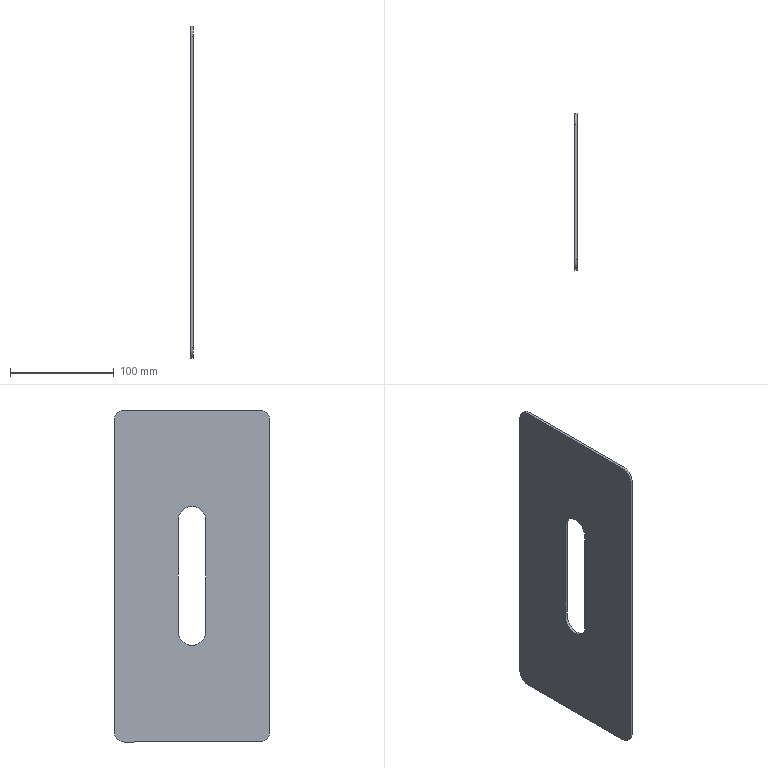Component | SolidWorks | 12ATransverseStraighteningSeatBaffle-1 | 1 solid | 15 faces | box 2.5 x 150.5 x 320.5 mm | volume 111720 mm3 | plane 8 | cylinder 7 | commonest cylinder face diameters 20 x4 27 x3 | material Q235
build123d program:
from build123d import *

# Parameters (mm, degrees)
BOSS_EXTRUDE1_DEPTH = 2.5


with BuildPart() as part:
    # Sketch1 → Boss-Extrude1 (new body)
    with BuildSketch(Plane.XY):
        with BuildLine():
            Line((-150.25, 75.25), (150.25, 75.25))
            ThreePointArc((150.25, 75.25), (157.321, 72.321), (160.25, 65.25))
            Line((160.25, 65.25), (160.25, -65.25))
            ThreePointArc((160.25, -65.25), (157.321, -72.321), (150.25, -75.25))
            Line((150.25, -75.25), (-150.25, -75.25))
            ThreePointArc((-150.25, -75.25), (-157.321, -72.321), (-160.25, -65.25))
            Line((-160.25, -65.25), (-160.25, 65.25))
            ThreePointArc((-160.25, 65.25), (-157.321, 72.321), (-150.25, 75.25))
        make_face()
        with BuildLine():
            Line((-53.5, 13.5), (53.5, 13.5))
            ThreePointArc((53.5, 13.5), (67, 0), (53.5, -13.5))
            Line((53.5, -13.5), (-53.5, -13.5))
            ThreePointArc((-53.5, -13.5), (-67, 0), (-53.5, 13.5))
        make_face(mode=Mode.SUBTRACT)
    extrude(amount=BOSS_EXTRUDE1_DEPTH)


solid = part.part

# Placed as in the assembly
solid = solid.moved(Location((-114.383, 6.96, 31), (0, 90, 0)))
STEP:
#1=COLOUR_RGB('',0.7922,0.8196,0.9333);
#2=FILL_AREA_STYLE_COLOUR('',#1);
#3=FILL_AREA_STYLE('',(#2));
#4=SURFACE_STYLE_FILL_AREA(#3);
#5=SURFACE_SIDE_STYLE('',(#4));
#6=SURFACE_STYLE_USAGE(.BOTH.,#5);
#7=PRESENTATION_STYLE_ASSIGNMENT((#6));
#8=CARTESIAN_POINT('',(-4.405,0.8055,3.327));
#9=VERTEX_POINT('',#8);
#10=CARTESIAN_POINT('',(-4.405,0.274,3.858));
#11=VERTEX_POINT('',#10);
#12=CARTESIAN_POINT('',(-4.405,0.274,3.327));
#13=DIRECTION('',(1.,0.,0.));
#14=DIRECTION('',(0.,-0.,-1.));
#15=AXIS2_PLACEMENT_3D('',#12,#13,#14);
#16=CIRCLE('',#15,0.5315);
#17=EDGE_CURVE('',#9,#11,#16,.T.);
#18=ORIENTED_EDGE('',*,*,#17,.T.);
#19=CARTESIAN_POINT('',(-4.503,0.274,3.858));
#20=VERTEX_POINT('',#19);
#21=CARTESIAN_POINT('',(-4.405,0.274,3.858));
#22=DIRECTION('',(-1.,-0.,0.));
#23=VECTOR('',#22,39.37);
#24=LINE('',#21,#23);
#25=EDGE_CURVE('',#11,#20,#24,.T.);
#26=ORIENTED_EDGE('',*,*,#25,.T.);
#27=CARTESIAN_POINT('',(-4.503,0.8055,3.327));
#28=VERTEX_POINT('',#27);
#29=CARTESIAN_POINT('',(-4.503,0.274,3.327));
#30=DIRECTION('',(1.,0.,0.));
#31=DIRECTION('',(0.,-0.,-1.));
#32=AXIS2_PLACEMENT_3D('',#29,#30,#31);
#33=CIRCLE('',#32,0.5315);
#34=EDGE_CURVE('',#28,#20,#33,.T.);
#35=ORIENTED_EDGE('',*,*,#34,.F.);
#36=CARTESIAN_POINT('',(-4.405,0.8055,3.327));
#37=DIRECTION('',(-1.,-0.,0.));
#38=VECTOR('',#37,39.37);
#39=LINE('',#36,#38);
#40=EDGE_CURVE('',#9,#28,#39,.T.);
#41=ORIENTED_EDGE('',*,*,#40,.F.);
#42=EDGE_LOOP('',(#18,#26,#35,#41));
#43=FACE_OUTER_BOUND('',#42,.T.);
#44=CARTESIAN_POINT('',(-4.405,0.274,3.327));
#45=DIRECTION('',(-1.,-0.,0.));
#46=DIRECTION('',(0.,0.,1.));
#47=AXIS2_PLACEMENT_3D('',#44,#45,#46);
#48=CYLINDRICAL_SURFACE('',#47,0.5315);
#49=ADVANCED_FACE('',(#43),#48,.F.);
#50=CARTESIAN_POINT('',(-4.405,2.843,-5.089));
#51=VERTEX_POINT('',#50);
#52=CARTESIAN_POINT('',(-4.405,3.237,-4.695));
#53=VERTEX_POINT('',#52);
#54=CARTESIAN_POINT('',(-4.405,2.843,-4.695));
#55=DIRECTION('',(1.,0.,0.));
#56=DIRECTION('',(0.,0.,1.));
#57=AXIS2_PLACEMENT_3D('',#54,#55,#56);
#58=CIRCLE('',#57,0.3937);
#59=EDGE_CURVE('',#51,#53,#58,.T.);
#60=ORIENTED_EDGE('',*,*,#59,.T.);
#61=CARTESIAN_POINT('',(-4.405,3.237,7.136));
#62=VERTEX_POINT('',#61);
#63=CARTESIAN_POINT('',(-4.405,3.237,7.136));
#64=DIRECTION('',(-0.,0.,1.));
#65=VECTOR('',#64,39.37);
#66=LINE('',#63,#65);
#67=EDGE_CURVE('',#53,#62,#66,.T.);
#68=ORIENTED_EDGE('',*,*,#67,.T.);
#69=CARTESIAN_POINT('',(-4.405,2.843,7.53));
#70=VERTEX_POINT('',#69);
#71=CARTESIAN_POINT('',(-4.405,2.843,7.136));
#72=DIRECTION('',(1.,0.,0.));
#73=DIRECTION('',(0.,-0.,-1.));
#74=AXIS2_PLACEMENT_3D('',#71,#72,#73);
#75=CIRCLE('',#74,0.3937);
#76=EDGE_CURVE('',#62,#70,#75,.T.);
#77=ORIENTED_EDGE('',*,*,#76,.T.);
#78=CARTESIAN_POINT('',(-4.405,-2.295,7.53));
#79=VERTEX_POINT('',#78);
#80=CARTESIAN_POINT('',(-4.405,2.843,7.53));
#81=DIRECTION('',(0.,-1.,0.));
#82=VECTOR('',#81,39.37);
#83=LINE('',#80,#82);
#84=EDGE_CURVE('',#70,#79,#83,.T.);
#85=ORIENTED_EDGE('',*,*,#84,.T.);
#86=CARTESIAN_POINT('',(-4.405,-2.689,7.136));
#87=VERTEX_POINT('',#86);
#88=CARTESIAN_POINT('',(-4.405,-2.295,7.136));
#89=DIRECTION('',(1.,0.,0.));
#90=DIRECTION('',(0.,-0.,-1.));
#91=AXIS2_PLACEMENT_3D('',#88,#89,#90);
#92=CIRCLE('',#91,0.3937);
#93=EDGE_CURVE('',#79,#87,#92,.T.);
#94=ORIENTED_EDGE('',*,*,#93,.T.);
#95=CARTESIAN_POINT('',(-4.405,-2.689,-4.695));
#96=VERTEX_POINT('',#95);
#97=CARTESIAN_POINT('',(-4.405,-2.689,7.136));
#98=DIRECTION('',(0.,-0.,-1.));
#99=VECTOR('',#98,39.37);
#100=LINE('',#97,#99);
#101=EDGE_CURVE('',#87,#96,#100,.T.);
#102=ORIENTED_EDGE('',*,*,#101,.T.);
#103=CARTESIAN_POINT('',(-4.405,-2.295,-5.089));
#104=VERTEX_POINT('',#103);
#105=CARTESIAN_POINT('',(-4.405,-2.295,-4.695));
#106=DIRECTION('',(1.,0.,0.));
#107=DIRECTION('',(0.,-0.,-1.));
#108=AXIS2_PLACEMENT_3D('',#105,#106,#107);
#109=CIRCLE('',#108,0.3937);
#110=EDGE_CURVE('',#96,#104,#109,.T.);
#111=ORIENTED_EDGE('',*,*,#110,.T.);
#112=CARTESIAN_POINT('',(-4.405,2.843,-5.089));
#113=DIRECTION('',(-0.,1.,-0.));
#114=VECTOR('',#113,39.37);
#115=LINE('',#112,#114);
#116=EDGE_CURVE('',#104,#51,#115,.T.);
#117=ORIENTED_EDGE('',*,*,#116,.T.);
#118=EDGE_LOOP('',(#60,#68,#77,#85,#94,#102,#111,#117));
#119=FACE_OUTER_BOUND('',#118,.T.);
#120=ORIENTED_EDGE('',*,*,#17,.F.);
#121=CARTESIAN_POINT('',(-4.405,0.8055,-0.8858));
#122=VERTEX_POINT('',#121);
#123=CARTESIAN_POINT('',(-4.405,0.8055,3.327));
#124=DIRECTION('',(-0.,0.,1.));
#125=VECTOR('',#124,39.37);
#126=LINE('',#123,#125);
#127=EDGE_CURVE('',#122,#9,#126,.T.);
#128=ORIENTED_EDGE('',*,*,#127,.F.);
#129=CARTESIAN_POINT('',(-4.405,-0.2575,-0.8858));
#130=VERTEX_POINT('',#129);
#131=CARTESIAN_POINT('',(-4.405,0.274,-0.8858));
#132=DIRECTION('',(1.,0.,0.));
#133=DIRECTION('',(0.,-0.,-1.));
#134=AXIS2_PLACEMENT_3D('',#131,#132,#133);
#135=CIRCLE('',#134,0.5315);
#136=EDGE_CURVE('',#130,#122,#135,.T.);
#137=ORIENTED_EDGE('',*,*,#136,.F.);
#138=CARTESIAN_POINT('',(-4.405,-0.2575,3.327));
#139=VERTEX_POINT('',#138);
#140=CARTESIAN_POINT('',(-4.405,-0.2575,3.327));
#141=DIRECTION('',(0.,-0.,-1.));
#142=VECTOR('',#141,39.37);
#143=LINE('',#140,#142);
#144=EDGE_CURVE('',#139,#130,#143,.T.);
#145=ORIENTED_EDGE('',*,*,#144,.F.);
#146=CARTESIAN_POINT('',(-4.405,0.274,3.327));
#147=DIRECTION('',(1.,0.,0.));
#148=DIRECTION('',(0.,-0.,-1.));
#149=AXIS2_PLACEMENT_3D('',#146,#147,#148);
#150=CIRCLE('',#149,0.5315);
#151=EDGE_CURVE('',#11,#139,#150,.T.);
#152=ORIENTED_EDGE('',*,*,#151,.F.);
#153=EDGE_LOOP('',(#120,#128,#137,#145,#152));
#154=FACE_BOUND('',#153,.T.);
#155=CARTESIAN_POINT('',(-4.405,2.843,-4.695));
#156=DIRECTION('',(-1.,-0.,-0.));
#157=DIRECTION('',(-0.,0.,1.));
#158=AXIS2_PLACEMENT_3D('',#155,#156,#157);
#159=PLANE('',#158);
#160=ADVANCED_FACE('',(#119,#154),#159,.F.);
#161=CARTESIAN_POINT('',(-4.503,2.843,-5.089));
#162=VERTEX_POINT('',#161);
#163=CARTESIAN_POINT('',(-4.503,3.237,-4.695));
#164=VERTEX_POINT('',#163);
#165=CARTESIAN_POINT('',(-4.503,2.843,-4.695));
#166=DIRECTION('',(1.,0.,0.));
#167=DIRECTION('',(0.,0.,1.));
#168=AXIS2_PLACEMENT_3D('',#165,#166,#167);
#169=CIRCLE('',#168,0.3937);
#170=EDGE_CURVE('',#162,#164,#169,.T.);
#171=ORIENTED_EDGE('',*,*,#170,.F.);
#172=CARTESIAN_POINT('',(-4.503,-2.295,-5.089));
#173=VERTEX_POINT('',#172);
#174=CARTESIAN_POINT('',(-4.503,2.843,-5.089));
#175=DIRECTION('',(-0.,1.,-0.));
#176=VECTOR('',#175,39.37);
#177=LINE('',#174,#176);
#178=EDGE_CURVE('',#173,#162,#177,.T.);
#179=ORIENTED_EDGE('',*,*,#178,.F.);
#180=CARTESIAN_POINT('',(-4.503,-2.689,-4.695));
#181=VERTEX_POINT('',#180);
#182=CARTESIAN_POINT('',(-4.503,-2.295,-4.695));
#183=DIRECTION('',(1.,0.,0.));
#184=DIRECTION('',(0.,-0.,-1.));
#185=AXIS2_PLACEMENT_3D('',#182,#183,#184);
#186=CIRCLE('',#185,0.3937);
#187=EDGE_CURVE('',#181,#173,#186,.T.);
#188=ORIENTED_EDGE('',*,*,#187,.F.);
#189=CARTESIAN_POINT('',(-4.503,-2.689,7.136));
#190=VERTEX_POINT('',#189);
#191=CARTESIAN_POINT('',(-4.503,-2.689,7.136));
#192=DIRECTION('',(0.,-0.,-1.));
#193=VECTOR('',#192,39.37);
#194=LINE('',#191,#193);
#195=EDGE_CURVE('',#190,#181,#194,.T.);
#196=ORIENTED_EDGE('',*,*,#195,.F.);
#197=CARTESIAN_POINT('',(-4.503,-2.295,7.53));
#198=VERTEX_POINT('',#197);
#199=CARTESIAN_POINT('',(-4.503,-2.295,7.136));
#200=DIRECTION('',(1.,0.,0.));
#201=DIRECTION('',(0.,-0.,-1.));
#202=AXIS2_PLACEMENT_3D('',#199,#200,#201);
#203=CIRCLE('',#202,0.3937);
#204=EDGE_CURVE('',#198,#190,#203,.T.);
#205=ORIENTED_EDGE('',*,*,#204,.F.);
#206=CARTESIAN_POINT('',(-4.503,2.843,7.53));
#207=VERTEX_POINT('',#206);
#208=CARTESIAN_POINT('',(-4.503,2.843,7.53));
#209=DIRECTION('',(0.,-1.,0.));
#210=VECTOR('',#209,39.37);
#211=LINE('',#208,#210);
#212=EDGE_CURVE('',#207,#198,#211,.T.);
#213=ORIENTED_EDGE('',*,*,#212,.F.);
#214=CARTESIAN_POINT('',(-4.503,3.237,7.136));
#215=VERTEX_POINT('',#214);
#216=CARTESIAN_POINT('',(-4.503,2.843,7.136));
#217=DIRECTION('',(1.,0.,0.));
#218=DIRECTION('',(0.,-0.,-1.));
#219=AXIS2_PLACEMENT_3D('',#216,#217,#218);
#220=CIRCLE('',#219,0.3937);
#221=EDGE_CURVE('',#215,#207,#220,.T.);
#222=ORIENTED_EDGE('',*,*,#221,.F.);
#223=CARTESIAN_POINT('',(-4.503,3.237,7.136));
#224=DIRECTION('',(-0.,0.,1.));
#225=VECTOR('',#224,39.37);
#226=LINE('',#223,#225);
#227=EDGE_CURVE('',#164,#215,#226,.T.);
#228=ORIENTED_EDGE('',*,*,#227,.F.);
#229=EDGE_LOOP('',(#171,#179,#188,#196,#205,#213,#222,#228));
#230=FACE_OUTER_BOUND('',#229,.T.);
#231=CARTESIAN_POINT('',(-4.503,0.8055,-0.8858));
#232=VERTEX_POINT('',#231);
#233=CARTESIAN_POINT('',(-4.503,0.8055,3.327));
#234=DIRECTION('',(-0.,0.,1.));
#235=VECTOR('',#234,39.37);
#236=LINE('',#233,#235);
#237=EDGE_CURVE('',#232,#28,#236,.T.);
#238=ORIENTED_EDGE('',*,*,#237,.T.);
#239=ORIENTED_EDGE('',*,*,#34,.T.);
#240=CARTESIAN_POINT('',(-4.503,-0.2575,3.327));
#241=VERTEX_POINT('',#240);
#242=CARTESIAN_POINT('',(-4.503,0.274,3.327));
#243=DIRECTION('',(1.,0.,0.));
#244=DIRECTION('',(0.,-0.,-1.));
#245=AXIS2_PLACEMENT_3D('',#242,#243,#244);
#246=CIRCLE('',#245,0.5315);
#247=EDGE_CURVE('',#20,#241,#246,.T.);
#248=ORIENTED_EDGE('',*,*,#247,.T.);
#249=CARTESIAN_POINT('',(-4.503,-0.2575,-0.8858));
#250=VERTEX_POINT('',#249);
#251=CARTESIAN_POINT('',(-4.503,-0.2575,3.327));
#252=DIRECTION('',(0.,-0.,-1.));
#253=VECTOR('',#252,39.37);
#254=LINE('',#251,#253);
#255=EDGE_CURVE('',#241,#250,#254,.T.);
#256=ORIENTED_EDGE('',*,*,#255,.T.);
#257=CARTESIAN_POINT('',(-4.503,0.274,-0.8858));
#258=DIRECTION('',(1.,0.,0.));
#259=DIRECTION('',(0.,-0.,-1.));
#260=AXIS2_PLACEMENT_3D('',#257,#258,#259);
#261=CIRCLE('',#260,0.5315);
#262=EDGE_CURVE('',#250,#232,#261,.T.);
#263=ORIENTED_EDGE('',*,*,#262,.T.);
#264=EDGE_LOOP('',(#238,#239,#248,#256,#263));
#265=FACE_BOUND('',#264,.T.);
#266=CARTESIAN_POINT('',(-4.503,2.843,-4.695));
#267=DIRECTION('',(-1.,-0.,-0.));
#268=DIRECTION('',(-0.,0.,1.));
#269=AXIS2_PLACEMENT_3D('',#266,#267,#268);
#270=PLANE('',#269);
#271=ADVANCED_FACE('',(#230,#265),#270,.T.);
#272=ORIENTED_EDGE('',*,*,#170,.T.);
#273=CARTESIAN_POINT('',(-4.405,3.237,-4.695));
#274=DIRECTION('',(-1.,-0.,0.));
#275=VECTOR('',#274,39.37);
#276=LINE('',#273,#275);
#277=EDGE_CURVE('',#53,#164,#276,.T.);
#278=ORIENTED_EDGE('',*,*,#277,.F.);
#279=ORIENTED_EDGE('',*,*,#59,.F.);
#280=CARTESIAN_POINT('',(-4.405,2.843,-5.089));
#281=DIRECTION('',(-1.,-0.,0.));
#282=VECTOR('',#281,39.37);
#283=LINE('',#280,#282);
#284=EDGE_CURVE('',#51,#162,#283,.T.);
#285=ORIENTED_EDGE('',*,*,#284,.T.);
#286=EDGE_LOOP('',(#272,#278,#279,#285));
#287=FACE_OUTER_BOUND('',#286,.T.);
#288=CARTESIAN_POINT('',(-4.405,2.843,-4.695));
#289=DIRECTION('',(-1.,-0.,0.));
#290=DIRECTION('',(0.,0.,1.));
#291=AXIS2_PLACEMENT_3D('',#288,#289,#290);
#292=CYLINDRICAL_SURFACE('',#291,0.3937);
#293=ADVANCED_FACE('',(#287),#292,.T.);
#294=ORIENTED_EDGE('',*,*,#227,.T.);
#295=CARTESIAN_POINT('',(-4.405,3.237,7.136));
#296=DIRECTION('',(-1.,-0.,0.));
#297=VECTOR('',#296,39.37);
#298=LINE('',#295,#297);
#299=EDGE_CURVE('',#62,#215,#298,.T.);
#300=ORIENTED_EDGE('',*,*,#299,.F.);
#301=ORIENTED_EDGE('',*,*,#67,.F.);
#302=ORIENTED_EDGE('',*,*,#277,.T.);
#303=EDGE_LOOP('',(#294,#300,#301,#302));
#304=FACE_OUTER_BOUND('',#303,.T.);
#305=CARTESIAN_POINT('',(-4.405,3.237,7.136));
#306=DIRECTION('',(0.,-1.,0.));
#307=DIRECTION('',(-1.,-0.,0.));
#308=AXIS2_PLACEMENT_3D('',#305,#306,#307);
#309=PLANE('',#308);
#310=ADVANCED_FACE('',(#304),#309,.F.);
#311=ORIENTED_EDGE('',*,*,#221,.T.);
#312=CARTESIAN_POINT('',(-4.405,2.843,7.53));
#313=DIRECTION('',(-1.,-0.,0.));
#314=VECTOR('',#313,39.37);
#315=LINE('',#312,#314);
#316=EDGE_CURVE('',#70,#207,#315,.T.);
#317=ORIENTED_EDGE('',*,*,#316,.F.);
#318=ORIENTED_EDGE('',*,*,#76,.F.);
#319=ORIENTED_EDGE('',*,*,#299,.T.);
#320=EDGE_LOOP('',(#311,#317,#318,#319));
#321=FACE_OUTER_BOUND('',#320,.T.);
#322=CARTESIAN_POINT('',(-4.405,2.843,7.136));
#323=DIRECTION('',(-1.,-0.,0.));
#324=DIRECTION('',(0.,0.,1.));
#325=AXIS2_PLACEMENT_3D('',#322,#323,#324);
#326=CYLINDRICAL_SURFACE('',#325,0.3937);
#327=ADVANCED_FACE('',(#321),#326,.T.);
#328=ORIENTED_EDGE('',*,*,#212,.T.);
#329=CARTESIAN_POINT('',(-4.405,-2.295,7.53));
#330=DIRECTION('',(-1.,-0.,0.));
#331=VECTOR('',#330,39.37);
#332=LINE('',#329,#331);
#333=EDGE_CURVE('',#79,#198,#332,.T.);
#334=ORIENTED_EDGE('',*,*,#333,.F.);
#335=ORIENTED_EDGE('',*,*,#84,.F.);
#336=ORIENTED_EDGE('',*,*,#316,.T.);
#337=EDGE_LOOP('',(#328,#334,#335,#336));
#338=FACE_OUTER_BOUND('',#337,.T.);
#339=CARTESIAN_POINT('',(-4.405,2.843,7.53));
#340=DIRECTION('',(0.,-0.,-1.));
#341=DIRECTION('',(-0.,1.,-0.));
#342=AXIS2_PLACEMENT_3D('',#339,#340,#341);
#343=PLANE('',#342);
#344=ADVANCED_FACE('',(#338),#343,.F.);
#345=ORIENTED_EDGE('',*,*,#204,.T.);
#346=CARTESIAN_POINT('',(-4.405,-2.689,7.136));
#347=DIRECTION('',(-1.,-0.,0.));
#348=VECTOR('',#347,39.37);
#349=LINE('',#346,#348);
#350=EDGE_CURVE('',#87,#190,#349,.T.);
#351=ORIENTED_EDGE('',*,*,#350,.F.);
#352=ORIENTED_EDGE('',*,*,#93,.F.);
#353=ORIENTED_EDGE('',*,*,#333,.T.);
#354=EDGE_LOOP('',(#345,#351,#352,#353));
#355=FACE_OUTER_BOUND('',#354,.T.);
#356=CARTESIAN_POINT('',(-4.405,-2.295,7.136));
#357=DIRECTION('',(-1.,-0.,0.));
#358=DIRECTION('',(0.,0.,1.));
#359=AXIS2_PLACEMENT_3D('',#356,#357,#358);
#360=CYLINDRICAL_SURFACE('',#359,0.3937);
#361=ADVANCED_FACE('',(#355),#360,.T.);
#362=ORIENTED_EDGE('',*,*,#195,.T.);
#363=CARTESIAN_POINT('',(-4.405,-2.689,-4.695));
#364=DIRECTION('',(-1.,-0.,0.));
#365=VECTOR('',#364,39.37);
#366=LINE('',#363,#365);
#367=EDGE_CURVE('',#96,#181,#366,.T.);
#368=ORIENTED_EDGE('',*,*,#367,.F.);
#369=ORIENTED_EDGE('',*,*,#101,.F.);
#370=ORIENTED_EDGE('',*,*,#350,.T.);
#371=EDGE_LOOP('',(#362,#368,#369,#370));
#372=FACE_OUTER_BOUND('',#371,.T.);
#373=CARTESIAN_POINT('',(-4.405,-2.689,7.136));
#374=DIRECTION('',(-0.,1.,-0.));
#375=DIRECTION('',(1.,0.,0.));
#376=AXIS2_PLACEMENT_3D('',#373,#374,#375);
#377=PLANE('',#376);
#378=ADVANCED_FACE('',(#372),#377,.F.);
#379=ORIENTED_EDGE('',*,*,#187,.T.);
#380=CARTESIAN_POINT('',(-4.405,-2.295,-5.089));
#381=DIRECTION('',(-1.,-0.,0.));
#382=VECTOR('',#381,39.37);
#383=LINE('',#380,#382);
#384=EDGE_CURVE('',#104,#173,#383,.T.);
#385=ORIENTED_EDGE('',*,*,#384,.F.);
#386=ORIENTED_EDGE('',*,*,#110,.F.);
#387=ORIENTED_EDGE('',*,*,#367,.T.);
#388=EDGE_LOOP('',(#379,#385,#386,#387));
#389=FACE_OUTER_BOUND('',#388,.T.);
#390=CARTESIAN_POINT('',(-4.405,-2.295,-4.695));
#391=DIRECTION('',(-1.,-0.,0.));
#392=DIRECTION('',(0.,0.,1.));
#393=AXIS2_PLACEMENT_3D('',#390,#391,#392);
#394=CYLINDRICAL_SURFACE('',#393,0.3937);
#395=ADVANCED_FACE('',(#389),#394,.T.);
#396=ORIENTED_EDGE('',*,*,#178,.T.);
#397=ORIENTED_EDGE('',*,*,#284,.F.);
#398=ORIENTED_EDGE('',*,*,#116,.F.);
#399=ORIENTED_EDGE('',*,*,#384,.T.);
#400=EDGE_LOOP('',(#396,#397,#398,#399));
#401=FACE_OUTER_BOUND('',#400,.T.);
#402=CARTESIAN_POINT('',(-4.405,2.843,-5.089));
#403=DIRECTION('',(-0.,0.,1.));
#404=DIRECTION('',(0.,-1.,0.));
#405=AXIS2_PLACEMENT_3D('',#402,#403,#404);
#406=PLANE('',#405);
#407=ADVANCED_FACE('',(#401),#406,.F.);
#408=ORIENTED_EDGE('',*,*,#25,.F.);
#409=ORIENTED_EDGE('',*,*,#151,.T.);
#410=CARTESIAN_POINT('',(-4.405,-0.2575,3.327));
#411=DIRECTION('',(-1.,-0.,0.));
#412=VECTOR('',#411,39.37);
#413=LINE('',#410,#412);
#414=EDGE_CURVE('',#139,#241,#413,.T.);
#415=ORIENTED_EDGE('',*,*,#414,.T.);
#416=ORIENTED_EDGE('',*,*,#247,.F.);
#417=EDGE_LOOP('',(#408,#409,#415,#416));
#418=FACE_OUTER_BOUND('',#417,.T.);
#419=CARTESIAN_POINT('',(-4.405,0.274,3.327));
#420=DIRECTION('',(-1.,-0.,0.));
#421=DIRECTION('',(0.,0.,1.));
#422=AXIS2_PLACEMENT_3D('',#419,#420,#421);
#423=CYLINDRICAL_SURFACE('',#422,0.5315);
#424=ADVANCED_FACE('',(#418),#423,.F.);
#425=ORIENTED_EDGE('',*,*,#255,.F.);
#426=ORIENTED_EDGE('',*,*,#414,.F.);
#427=ORIENTED_EDGE('',*,*,#144,.T.);
#428=CARTESIAN_POINT('',(-4.405,-0.2575,-0.8858));
#429=DIRECTION('',(-1.,-0.,0.));
#430=VECTOR('',#429,39.37);
#431=LINE('',#428,#430);
#432=EDGE_CURVE('',#130,#250,#431,.T.);
#433=ORIENTED_EDGE('',*,*,#432,.T.);
#434=EDGE_LOOP('',(#425,#426,#427,#433));
#435=FACE_OUTER_BOUND('',#434,.T.);
#436=CARTESIAN_POINT('',(-4.405,-0.2575,3.327));
#437=DIRECTION('',(-0.,1.,-0.));
#438=DIRECTION('',(-0.,0.,1.));
#439=AXIS2_PLACEMENT_3D('',#436,#437,#438);
#440=PLANE('',#439);
#441=ADVANCED_FACE('',(#435),#440,.T.);
#442=ORIENTED_EDGE('',*,*,#262,.F.);
#443=ORIENTED_EDGE('',*,*,#432,.F.);
#444=ORIENTED_EDGE('',*,*,#136,.T.);
#445=CARTESIAN_POINT('',(-4.405,0.8055,-0.8858));
#446=DIRECTION('',(-1.,-0.,0.));
#447=VECTOR('',#446,39.37);
#448=LINE('',#445,#447);
#449=EDGE_CURVE('',#122,#232,#448,.T.);
#450=ORIENTED_EDGE('',*,*,#449,.T.);
#451=EDGE_LOOP('',(#442,#443,#444,#450));
#452=FACE_OUTER_BOUND('',#451,.T.);
#453=CARTESIAN_POINT('',(-4.405,0.274,-0.8858));
#454=DIRECTION('',(-1.,-0.,0.));
#455=DIRECTION('',(0.,0.,1.));
#456=AXIS2_PLACEMENT_3D('',#453,#454,#455);
#457=CYLINDRICAL_SURFACE('',#456,0.5315);
#458=ADVANCED_FACE('',(#452),#457,.F.);
#459=ORIENTED_EDGE('',*,*,#237,.F.);
#460=ORIENTED_EDGE('',*,*,#449,.F.);
#461=ORIENTED_EDGE('',*,*,#127,.T.);
#462=ORIENTED_EDGE('',*,*,#40,.T.);
#463=EDGE_LOOP('',(#459,#460,#461,#462));
#464=FACE_OUTER_BOUND('',#463,.T.);
#465=CARTESIAN_POINT('',(-4.405,0.8055,3.327));
#466=DIRECTION('',(0.,-1.,0.));
#467=DIRECTION('',(0.,-0.,-1.));
#468=AXIS2_PLACEMENT_3D('',#465,#466,#467);
#469=PLANE('',#468);
#470=ADVANCED_FACE('',(#464),#469,.T.);
#471=CLOSED_SHELL('',(#49,#160,#271,#293,#310,#327,#344,#361,#378,#395,#407,#424,#441,#458,#470));
#472=MANIFOLD_SOLID_BREP('',#471);
#473=STYLED_ITEM('',(#7),#472);
#474=(LENGTH_UNIT()NAMED_UNIT(*)SI_UNIT($,.METRE.));
#475=LENGTH_MEASURE_WITH_UNIT(LENGTH_MEASURE(0.0254),#474);
#476=DIMENSIONAL_EXPONENTS(1.,0.,0.,0.,0.,0.,0.);
#477=(CONVERSION_BASED_UNIT('',#475)LENGTH_UNIT()NAMED_UNIT(#476));
#478=UNCERTAINTY_MEASURE_WITH_UNIT(LENGTH_MEASURE(0.00001),#477,'','');
#479=(NAMED_UNIT(*)PLANE_ANGLE_UNIT()SI_UNIT($,.RADIAN.));
#480=(NAMED_UNIT(*)SI_UNIT($,.STERADIAN.)SOLID_ANGLE_UNIT());
#481=(GEOMETRIC_REPRESENTATION_CONTEXT(3)GLOBAL_UNCERTAINTY_ASSIGNED_CONTEXT((#478))GLOBAL_UNIT_ASSIGNED_CONTEXT((#477,#479,#480))REPRESENTATION_CONTEXT('',''));
#482=MECHANICAL_DESIGN_GEOMETRIC_PRESENTATION_REPRESENTATION('',(#473),#481);
#483=PRESENTATION_LAYER_ASSIGNMENT('','',(#473));
#484=CARTESIAN_POINT('',(0.,0.,0.));
#485=DIRECTION('',(0.,0.,1.));
#486=DIRECTION('',(1.,0.,0.));
#487=AXIS2_PLACEMENT_3D('',#484,#485,#486);
#488=(LENGTH_UNIT()NAMED_UNIT(*)SI_UNIT($,.METRE.));
#489=LENGTH_MEASURE_WITH_UNIT(LENGTH_MEASURE(0.0254),#488);
#490=DIMENSIONAL_EXPONENTS(1.,0.,0.,0.,0.,0.,0.);
#491=(CONVERSION_BASED_UNIT('',#489)LENGTH_UNIT()NAMED_UNIT(#490));
#492=UNCERTAINTY_MEASURE_WITH_UNIT(LENGTH_MEASURE(0.00001),#491,'','');
#493=(NAMED_UNIT(*)PLANE_ANGLE_UNIT()SI_UNIT($,.RADIAN.));
#494=(NAMED_UNIT(*)SI_UNIT($,.STERADIAN.)SOLID_ANGLE_UNIT());
#495=(GEOMETRIC_REPRESENTATION_CONTEXT(3)GLOBAL_UNCERTAINTY_ASSIGNED_CONTEXT((#492))GLOBAL_UNIT_ASSIGNED_CONTEXT((#491,#493,#494))REPRESENTATION_CONTEXT('',''));
#496=ADVANCED_BREP_SHAPE_REPRESENTATION('',(#472,#487),#495);